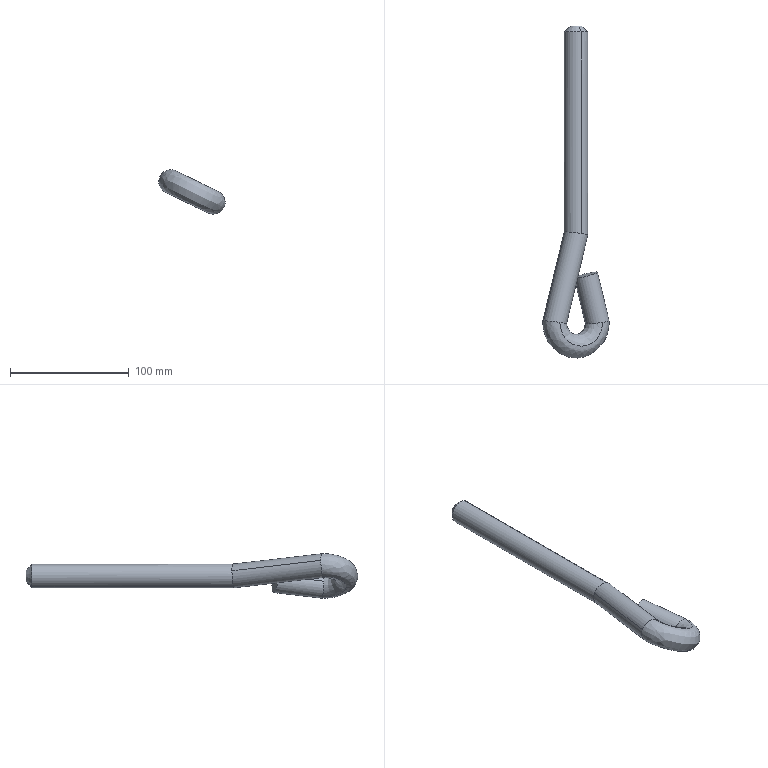Component | SolidWorks | JB_ZQ4363-2006AnchorBoltTypeA20_630-2 | 1 solid | 12 faces | volume 111445 mm3 | cylinder 6 | cone 2 | spline 2 | plane 2 | commonest cylinder face diameters 20 x6